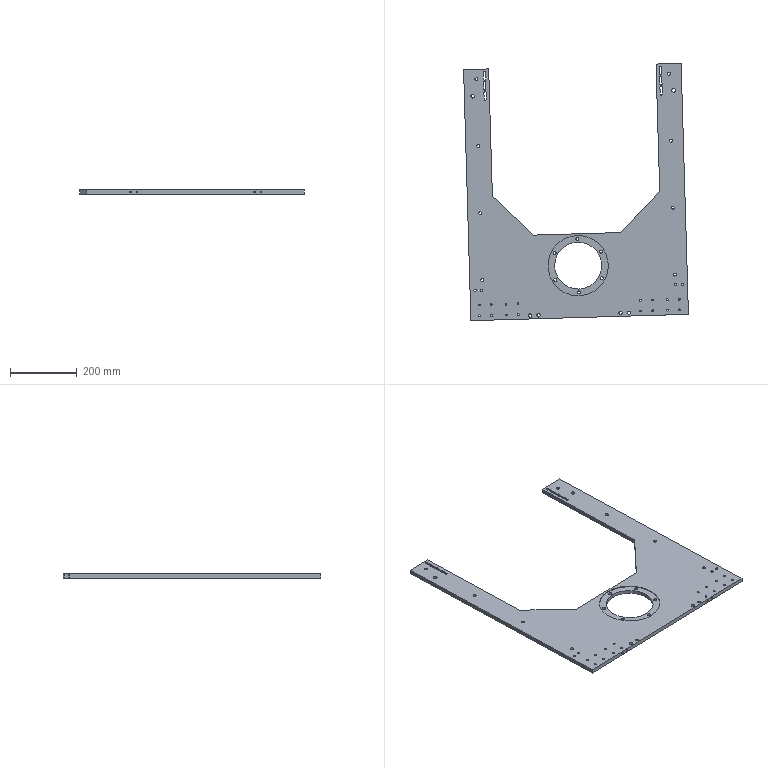Component | SolidWorks | RotatingPlatform-1 | 1 solid | 203 faces | box 671.61 x 768.65 x 12 mm | volume 2771625 mm3 | cylinder 148 | plane 47 | cone 8 | commonest cylinder face diameters 10 x40 5.5 x32 9 x28 6.5 x18 5 x8 6.8 x8 10.5 x6 11 x4 | material 6063
build123d program:
from build123d import *

# Parameters (mm, degrees)
SKETCH1_W                                       = 750
SKETCH1_H                                       = 650
BOSS_EXTRUDE1_DEPTH                             = 6
SKETCH2_R                                       = 5.5
CUT_EXTRUDE1_DEPTH                              = 497.381
M8_TAPPED_HOLE1_D                               = 6.8
M8_TAPPED_HOLE1_DEPTH                           = 19.75
M8_TAPPED_HOLE1_TIP                             = 2.043
M5_HEX_SOCKET_HEAD_CAP_SCREW_CBORE1_D           = 5.5
M5_HEX_SOCKET_HEAD_CAP_SCREW_CBORE1_CBORE_D     = 10
M5_HEX_SOCKET_HEAD_CAP_SCREW_CBORE1_CBORE_DEPTH = 5.4
SKETCH8_R                                       = 5
CUT_EXTRUDE2_DEPTH                              = 497.381
M6_TAPPED_HOLE2_AT_2_COUNT                      = 2
M6_TAPPED_HOLE2_AT_2_PITCH                      = 20
SKETCH14_R                                      = 90
CUT_EXTRUDE3_DEPTH                              = 2
SKETCH15_R                                      = 70
CUT_EXTRUDE4_DEPTH                              = 497.337
SKETCH16_R                                      = 4.5
CUT_EXTRUDE5_DEPTH                              = 497.381
SKETCH18_W                                      = 1000
SKETCH18_H                                      = 500
CUT_EXTRUDE6_DEPTH                              = 497.381
CHAMFER1_SIZE                                   = 120
F_9_0_9_DIAMETER_HOLE1_AT_2_COUNT               = 2
F_9_0_9_DIAMETER_HOLE1_AT_2_PITCH               = 575
LPATTERN1_COUNT                                 = 4
LPATTERN1_PITCH                                 = 200
CUT_EXTRUDE7_DEPTH                              = 497.381
LPATTERN2_COUNT                                 = 3
LPATTERN2_PITCH                                 = 30
CUT_EXTRUDE8_DEPTH                              = 6.5


with BuildPart() as part:
    # Sketch1 → Boss-Extrude1 (new, symmetric)
    with BuildSketch(Plane.XY):
        Rectangle(SKETCH1_W, SKETCH1_H)
    extrude(amount=BOSS_EXTRUDE1_DEPTH, both=True)

    # Sketch2 → Cut-Extrude1 (cut, through all)
    with BuildSketch(Plane.XY.offset(6)):
        with Locations((295, 300)):
            Circle(SKETCH2_R)
        with Locations((295, -300)):
            Circle(SKETCH2_R)
    extrude(amount=-CUT_EXTRUDE1_DEPTH, mode=Mode.SUBTRACT)

    # M8 Tapped Hole1
    with Locations(Plane(origin=(-285, 310, 6), x_dir=(1, 0, 0), z_dir=(0, 0, 1))):
        with Locations((0, 0), (0, -20), (0, -600), (0, -620)):
            Hole(M8_TAPPED_HOLE1_D / 2, depth=M8_TAPPED_HOLE1_DEPTH)
            with Locations((0, 0, -(M8_TAPPED_HOLE1_DEPTH + M8_TAPPED_HOLE1_TIP / 2))):  # 118° drill point
                Cone(0, M8_TAPPED_HOLE1_D / 2, M8_TAPPED_HOLE1_TIP, mode=Mode.SUBTRACT)

    # M5 Hex Socket Head Cap Screw CBORE1 (through all)
    with Locations(Plane(origin=(-329, -183, 6), x_dir=(1, 0, 0), z_dir=(0, 0, 1))):
        with Locations((0, 0), (-32, 0), (-32, -36), (0, -36), (0, -80), (0, -116), (-32, -116), (-32, -80)):
            m5_hex_socket_head_cap_screw_cbore1 = CounterBoreHole(M5_HEX_SOCKET_HEAD_CAP_SCREW_CBORE1_D / 2, M5_HEX_SOCKET_HEAD_CAP_SCREW_CBORE1_CBORE_D / 2, M5_HEX_SOCKET_HEAD_CAP_SCREW_CBORE1_CBORE_DEPTH)

    # Sketch8 → Cut-Extrude2 (cut, through all)
    with BuildSketch(Plane.XY.offset(6)):
        with Locations((-365, -122.5)):
            Circle(SKETCH8_R)
        with Locations((-365, -147.5)):
            Circle(SKETCH8_R)
    cut_extrude2 = extrude(amount=-CUT_EXTRUDE2_DEPTH, mode=Mode.SUBTRACT)

    # Mirror1: M5 Hex Socket Head Cap Screw CBORE1, Cut-Extrude2 across plane
    add(m5_hex_socket_head_cap_screw_cbore1.mirror(Plane.ZX), mode=Mode.SUBTRACT)
    add(cut_extrude2.mirror(Plane.ZX), mode=Mode.SUBTRACT)

    # Sketch12 → M6 Tapped Hole2 (revolve, cut)
    with BuildSketch(Plane(origin=(-375, 195, 0), x_dir=(0, 0, 1), z_dir=(0, 1, 0))):
        Polygon((0, 0), (0, 16.502), (2.5, 15), (2.5, 0), align=None)
    m6_tapped_hole2 = revolve(axis=Axis((-381.35, 195, 0), (1, 0, 0)), mode=Mode.SUBTRACT)

    # M6 Tapped Hole2 at 2: M6 Tapped Hole2 ×2
    with Locations(*[(0, -i * M6_TAPPED_HOLE2_AT_2_PITCH, 0) for i in range(1, M6_TAPPED_HOLE2_AT_2_COUNT)]):
        add(m6_tapped_hole2, mode=Mode.SUBTRACT)

    # Mirror3: M6 Tapped Hole2 across plane
    add(m6_tapped_hole2.mirror(Plane.ZX), mode=Mode.SUBTRACT)

    # Mirror3 copy 1 sketch → Mirror3 copy 1 (revolve, cut)
    with BuildSketch(Plane(origin=(-375, -175, 0), x_dir=(0, 0, 1), z_dir=(0, -1, 0))):
        Polygon((0, 0), (0, -16.502), (2.5, -15), (2.5, 0), align=None)
    revolve(axis=Axis((-381.35, -175, 0), (-1, 0, 0)), mode=Mode.SUBTRACT)

    # Sketch14 → Cut-Extrude3 (cut)
    with BuildSketch(Plane(origin=(0, 0, -6), x_dir=(-1, 0, 0), z_dir=(0, 0, -1))):
        with Locations((220, 0)):
            Circle(SKETCH14_R)
    extrude(amount=-CUT_EXTRUDE3_DEPTH, mode=Mode.SUBTRACT)

    # Sketch15 → Cut-Extrude4 (cut, through all)
    with BuildSketch(Plane(origin=(0, 0, -4), x_dir=(-1, 0, 0), z_dir=(0, 0, -1))):
        with Locations((220, 0)):
            Circle(SKETCH15_R)
    extrude(amount=-CUT_EXTRUDE4_DEPTH, mode=Mode.SUBTRACT)

    # Sketch16 → Cut-Extrude5 (cut, through all)
    with BuildSketch(Plane.XY.offset(6)):
        with Locations((-260, 69.282)):
            Circle(SKETCH16_R)
        with Locations((-180, 69.282)):
            Circle(SKETCH16_R)
        with Locations((-140, 0)):
            Circle(SKETCH16_R)
        with Locations((-180, -69.282)):
            Circle(SKETCH16_R)
        with Locations((-260, -69.282)):
            Circle(SKETCH16_R)
        with Locations((-300, 0)):
            Circle(SKETCH16_R)
    extrude(amount=-CUT_EXTRUDE5_DEPTH, mode=Mode.SUBTRACT)

    # Sketch18 → Cut-Extrude6 (cut, through all)
    with BuildSketch(Plane.XY.offset(6)):
        with Locations((375, 0)):
            Rectangle(SKETCH18_W, SKETCH18_H)
    extrude(amount=-CUT_EXTRUDE6_DEPTH, mode=Mode.SUBTRACT)

    # Chamfer1
    chamfer1_edges = [part.edges().sort_by_distance(p)[0] for p in [
        (-125, 250, 0),
        (-125, -250, 0),
    ]]
    chamfer(chamfer1_edges, length=CHAMFER1_SIZE)

    # Sketch21 → 9.0 _9_ Diameter Hole1 (revolve, cut)
    with BuildSketch(Plane(origin=(345, 287.5, 6), x_dir=(0, -1, 0), z_dir=(1, 0, 0))):
        Polygon((0, 0), (0, 102.598), (4.5, 100), (4.5, 0), align=None)
    f_9_0_9_diameter_hole1 = revolve(axis=Axis((345, 287.5, 12.35), (0, 0, -1)), mode=Mode.SUBTRACT)

    # 9.0 _9_ Diameter Hole1 at 2: 9.0 _9_ Diameter Hole1 ×2
    with Locations(*[(0, -i * F_9_0_9_DIAMETER_HOLE1_AT_2_PITCH, 0) for i in range(1, F_9_0_9_DIAMETER_HOLE1_AT_2_COUNT)]):
        add(f_9_0_9_diameter_hole1, mode=Mode.SUBTRACT)

    # LPattern1: 9.0 _9_ Diameter Hole1 ×4
    with Locations(*[(-i * LPATTERN1_PITCH, 0, 0) for i in range(1, LPATTERN1_COUNT)]):
        add(f_9_0_9_diameter_hole1, mode=Mode.SUBTRACT)

    # LPattern1 copy 1 sketch → LPattern1 copy 1 (revolve, cut)
    with BuildSketch(Plane(origin=(145, -287.5, 6), x_dir=(0, -1, 0), z_dir=(1, 0, 0))):
        Polygon((0, 0), (0, 102.598), (4.5, 100), (4.5, 0), align=None)
    revolve(axis=Axis((145, -287.5, 12.35), (0, 0, -1)), mode=Mode.SUBTRACT)

    # LPattern1 copy 2 sketch → LPattern1 copy 2 (revolve, cut)
    with BuildSketch(Plane(origin=(-55, -287.5, 6), x_dir=(0, -1, 0), z_dir=(1, 0, 0))):
        Polygon((0, 0), (0, 102.598), (4.5, 100), (4.5, 0), align=None)
    revolve(axis=Axis((-55, -287.5, 12.35), (0, 0, -1)), mode=Mode.SUBTRACT)

    # LPattern1 copy 3 sketch → LPattern1 copy 3 (revolve, cut)
    with BuildSketch(Plane(origin=(-255, -287.5, 6), x_dir=(0, -1, 0), z_dir=(1, 0, 0))):
        Polygon((0, 0), (0, 102.598), (4.5, 100), (4.5, 0), align=None)
    revolve(axis=Axis((-255, -287.5, 12.35), (0, 0, -1)), mode=Mode.SUBTRACT)

    # Sketch22 → Cut-Extrude7 (cut, through all)
    with BuildSketch(Plane.XY.offset(6)):
        with BuildLine():
            Line((365, 259.75), (345, 259.75))
            ThreePointArc((345, 259.75), (341.75, 263), (345, 266.25))
            Line((345, 266.25), (365, 266.25))
            ThreePointArc((365, 266.25), (368.25, 263), (365, 259.75))
        make_face()
        with BuildLine():
            Line((365, -259.75), (345, -259.75))
            ThreePointArc((345, -259.75), (341.75, -263), (345, -266.25))
            Line((345, -266.25), (365, -266.25))
            ThreePointArc((365, -266.25), (368.25, -263), (365, -259.75))
        make_face()
    cut_extrude7 = extrude(amount=-CUT_EXTRUDE7_DEPTH, mode=Mode.SUBTRACT)

    # LPattern2: Cut-Extrude7 ×3
    with Locations(*[(-i * LPATTERN2_PITCH, 0, 0) for i in range(1, LPATTERN2_COUNT)]):
        add(cut_extrude7, mode=Mode.SUBTRACT)

    # Sketch23 → Cut-Extrude8 (cut)
    with BuildSketch(Plane.XY.offset(6)):
        with BuildLine():
            Line((282.5, 268.25), (367.5, 268.25))
            ThreePointArc((367.5, 268.25), (372.75, 263), (367.5, 257.75))
            Line((367.5, 257.75), (282.5, 257.75))
            ThreePointArc((282.5, 257.75), (277.25, 263), (282.5, 268.25))
        make_face()
        with BuildLine():
            Line((282.5, -257.75), (367.5, -257.75))
            ThreePointArc((367.5, -257.75), (372.75, -263), (367.5, -268.25))
            Line((367.5, -268.25), (282.5, -268.25))
            ThreePointArc((282.5, -268.25), (277.25, -263), (282.5, -257.75))
        make_face()
    extrude(amount=-CUT_EXTRUDE8_DEPTH, mode=Mode.SUBTRACT)


solid = part.part

# Placed as in the assembly
solid = solid.moved(Location((-4.636, 192.989, -1268.21), (180, 0, -91.672)))